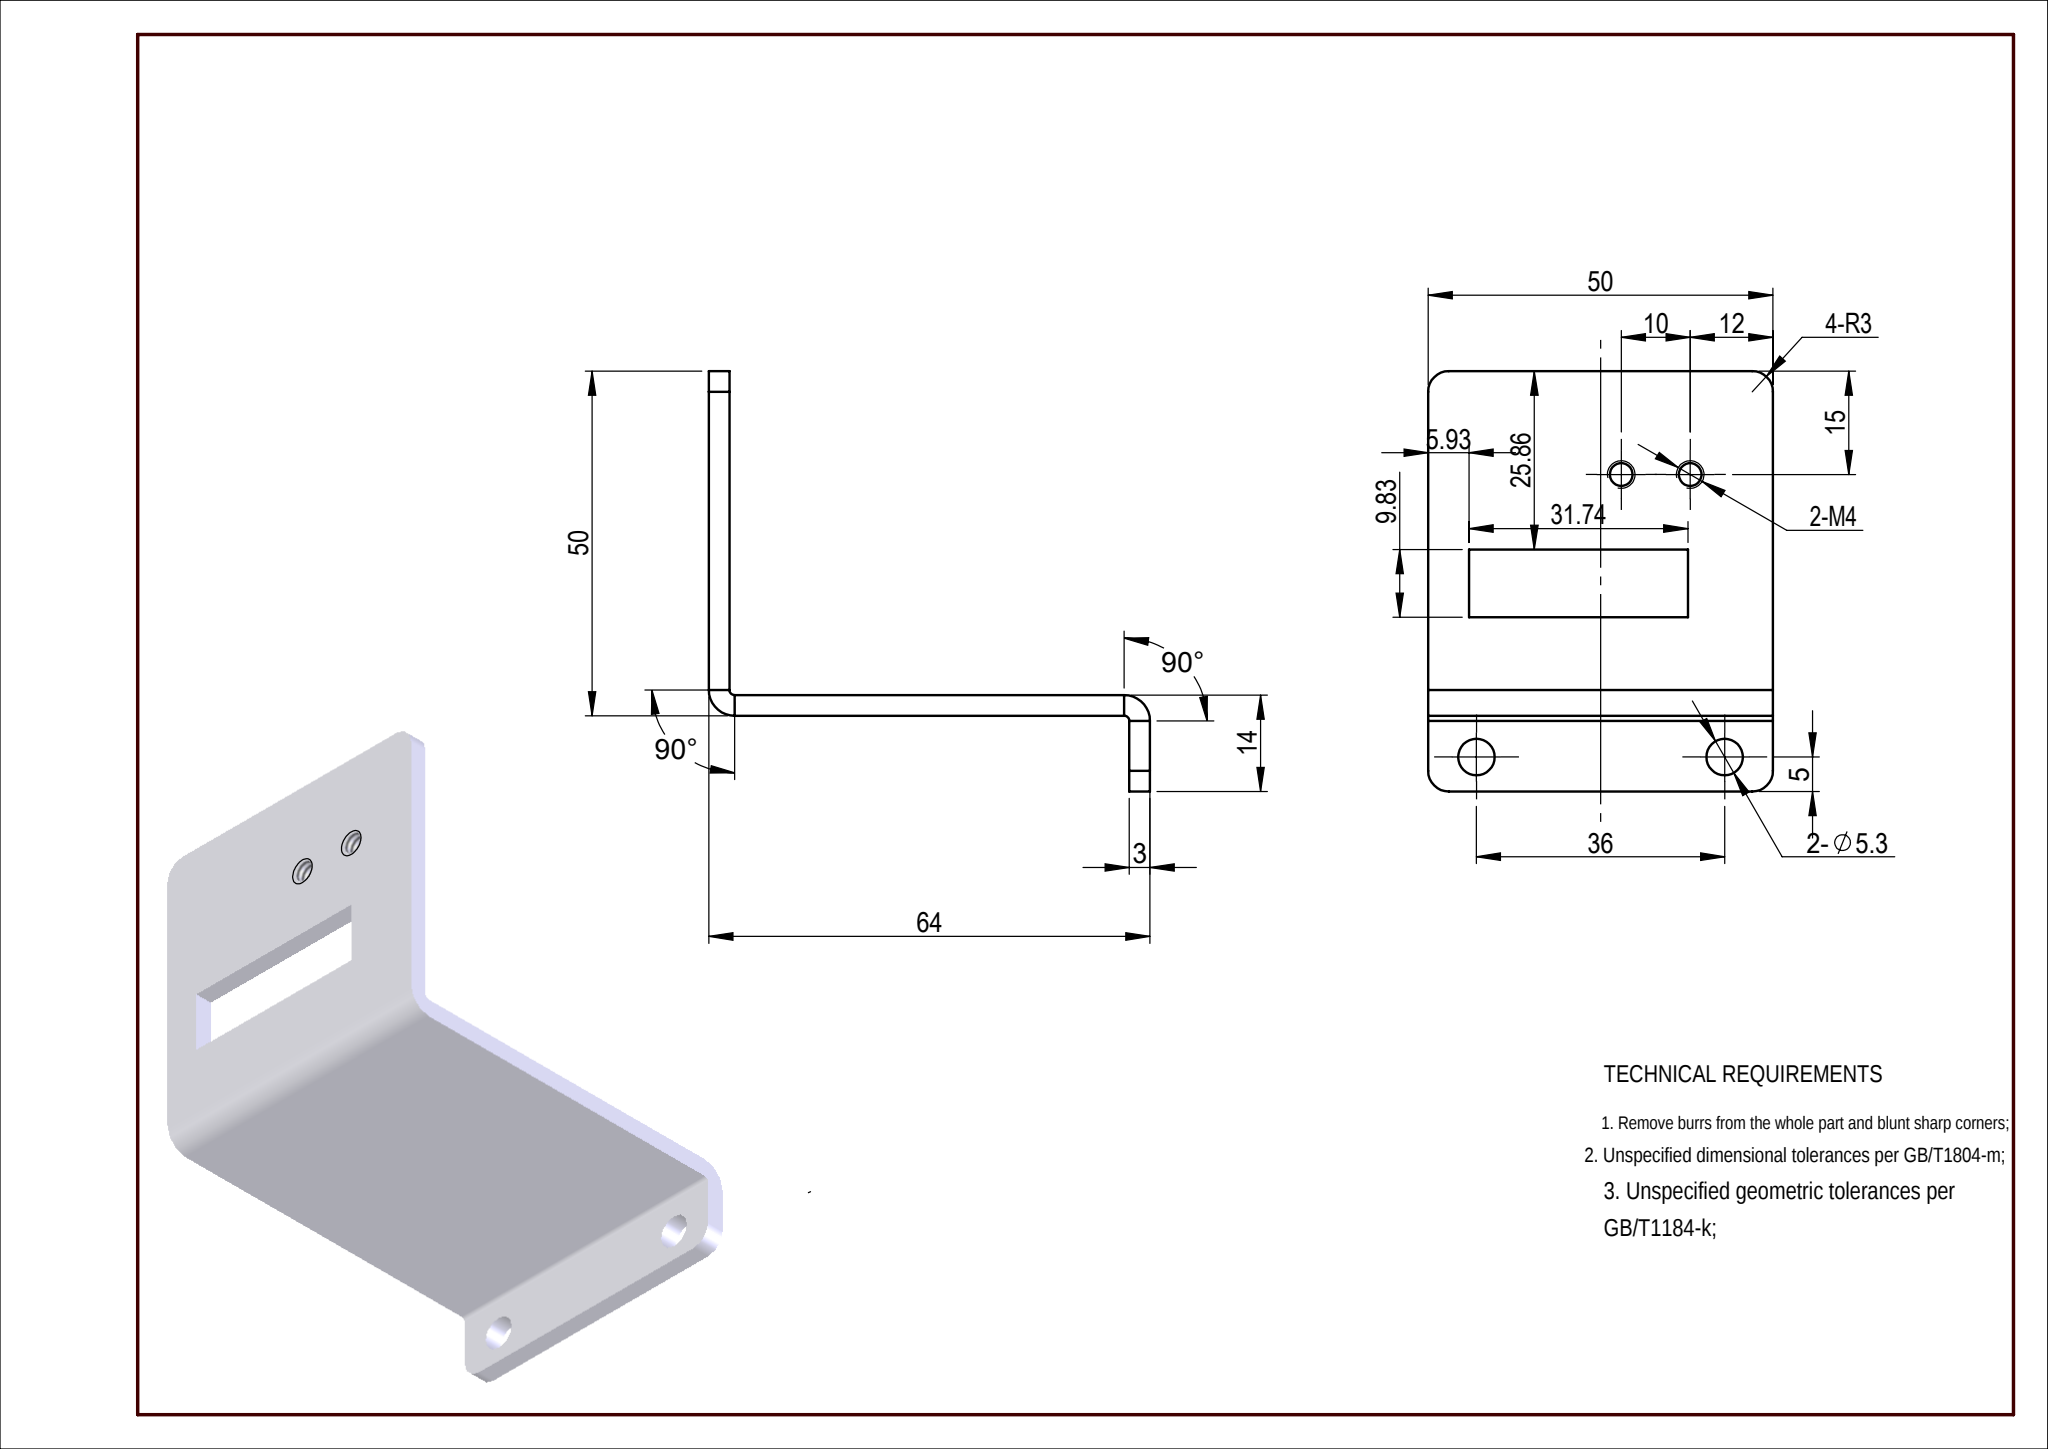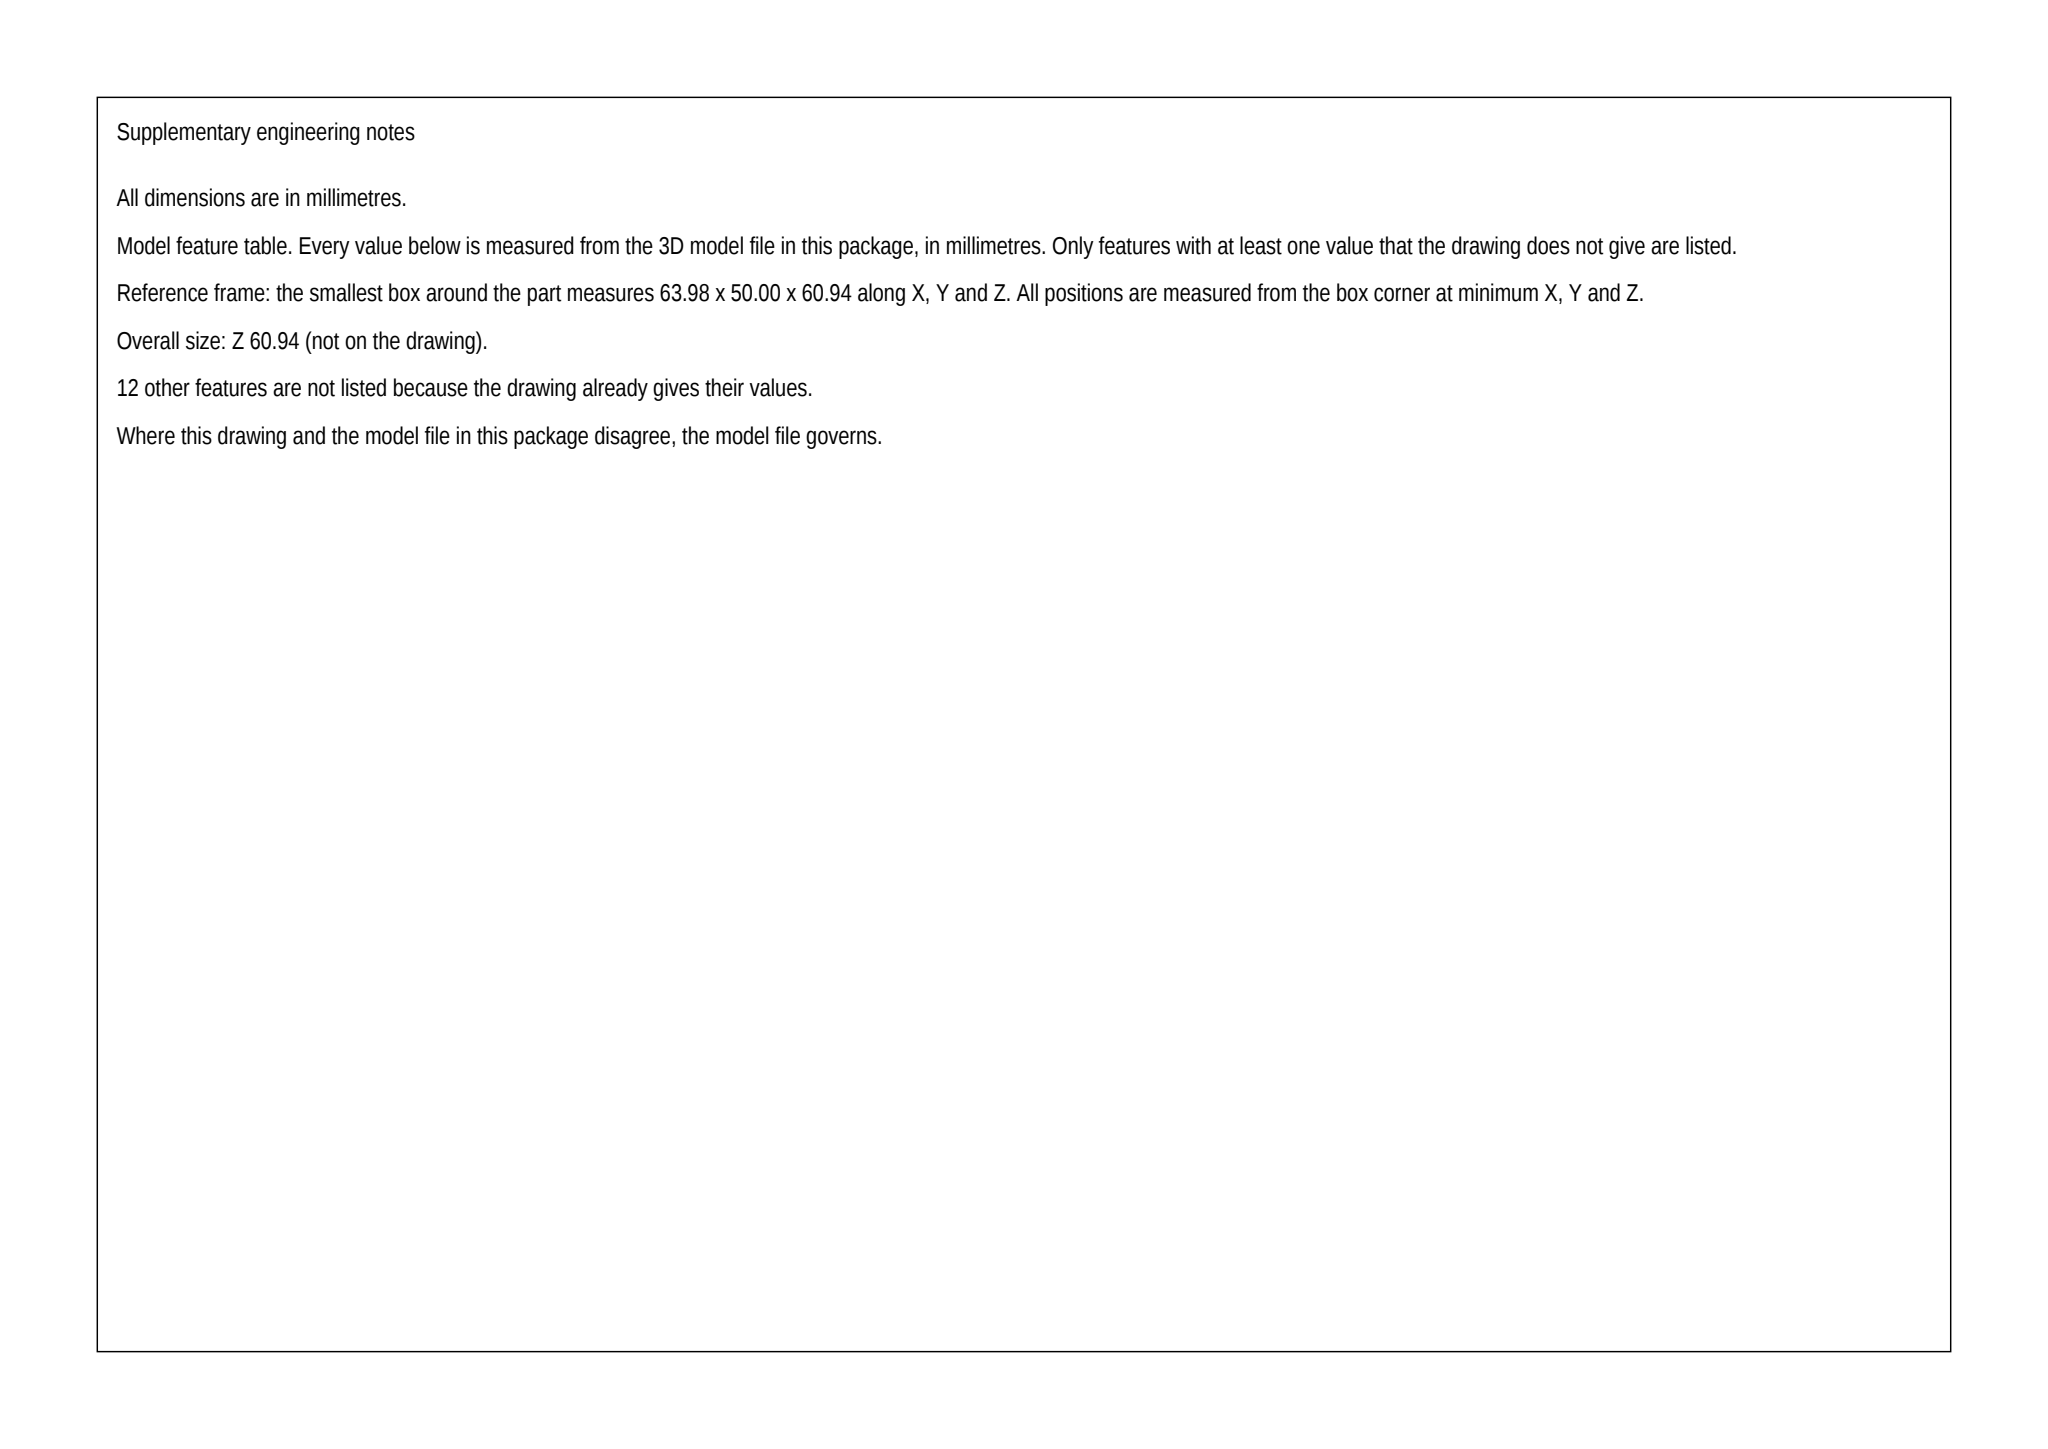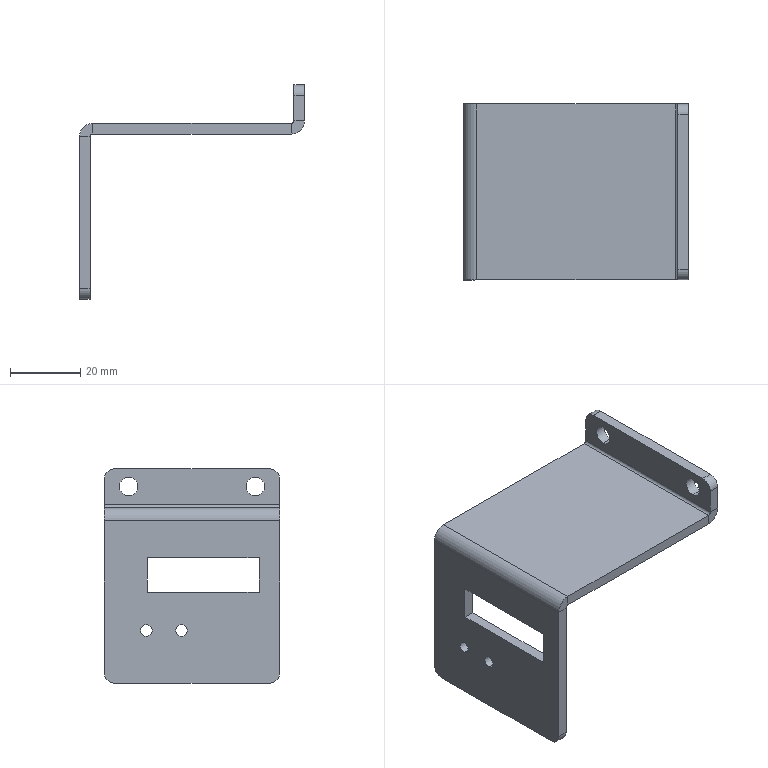Part | SolidWorks | mm | 1 solid | 38 faces | box 63.98 x 50 x 60.94 mm | volume 16857 mm3 | plane 22 | cylinder 16 | commonest cylinder face diameters 3.3 x4 5.3 x4 6 x4 7.473 x2 1.473 x2